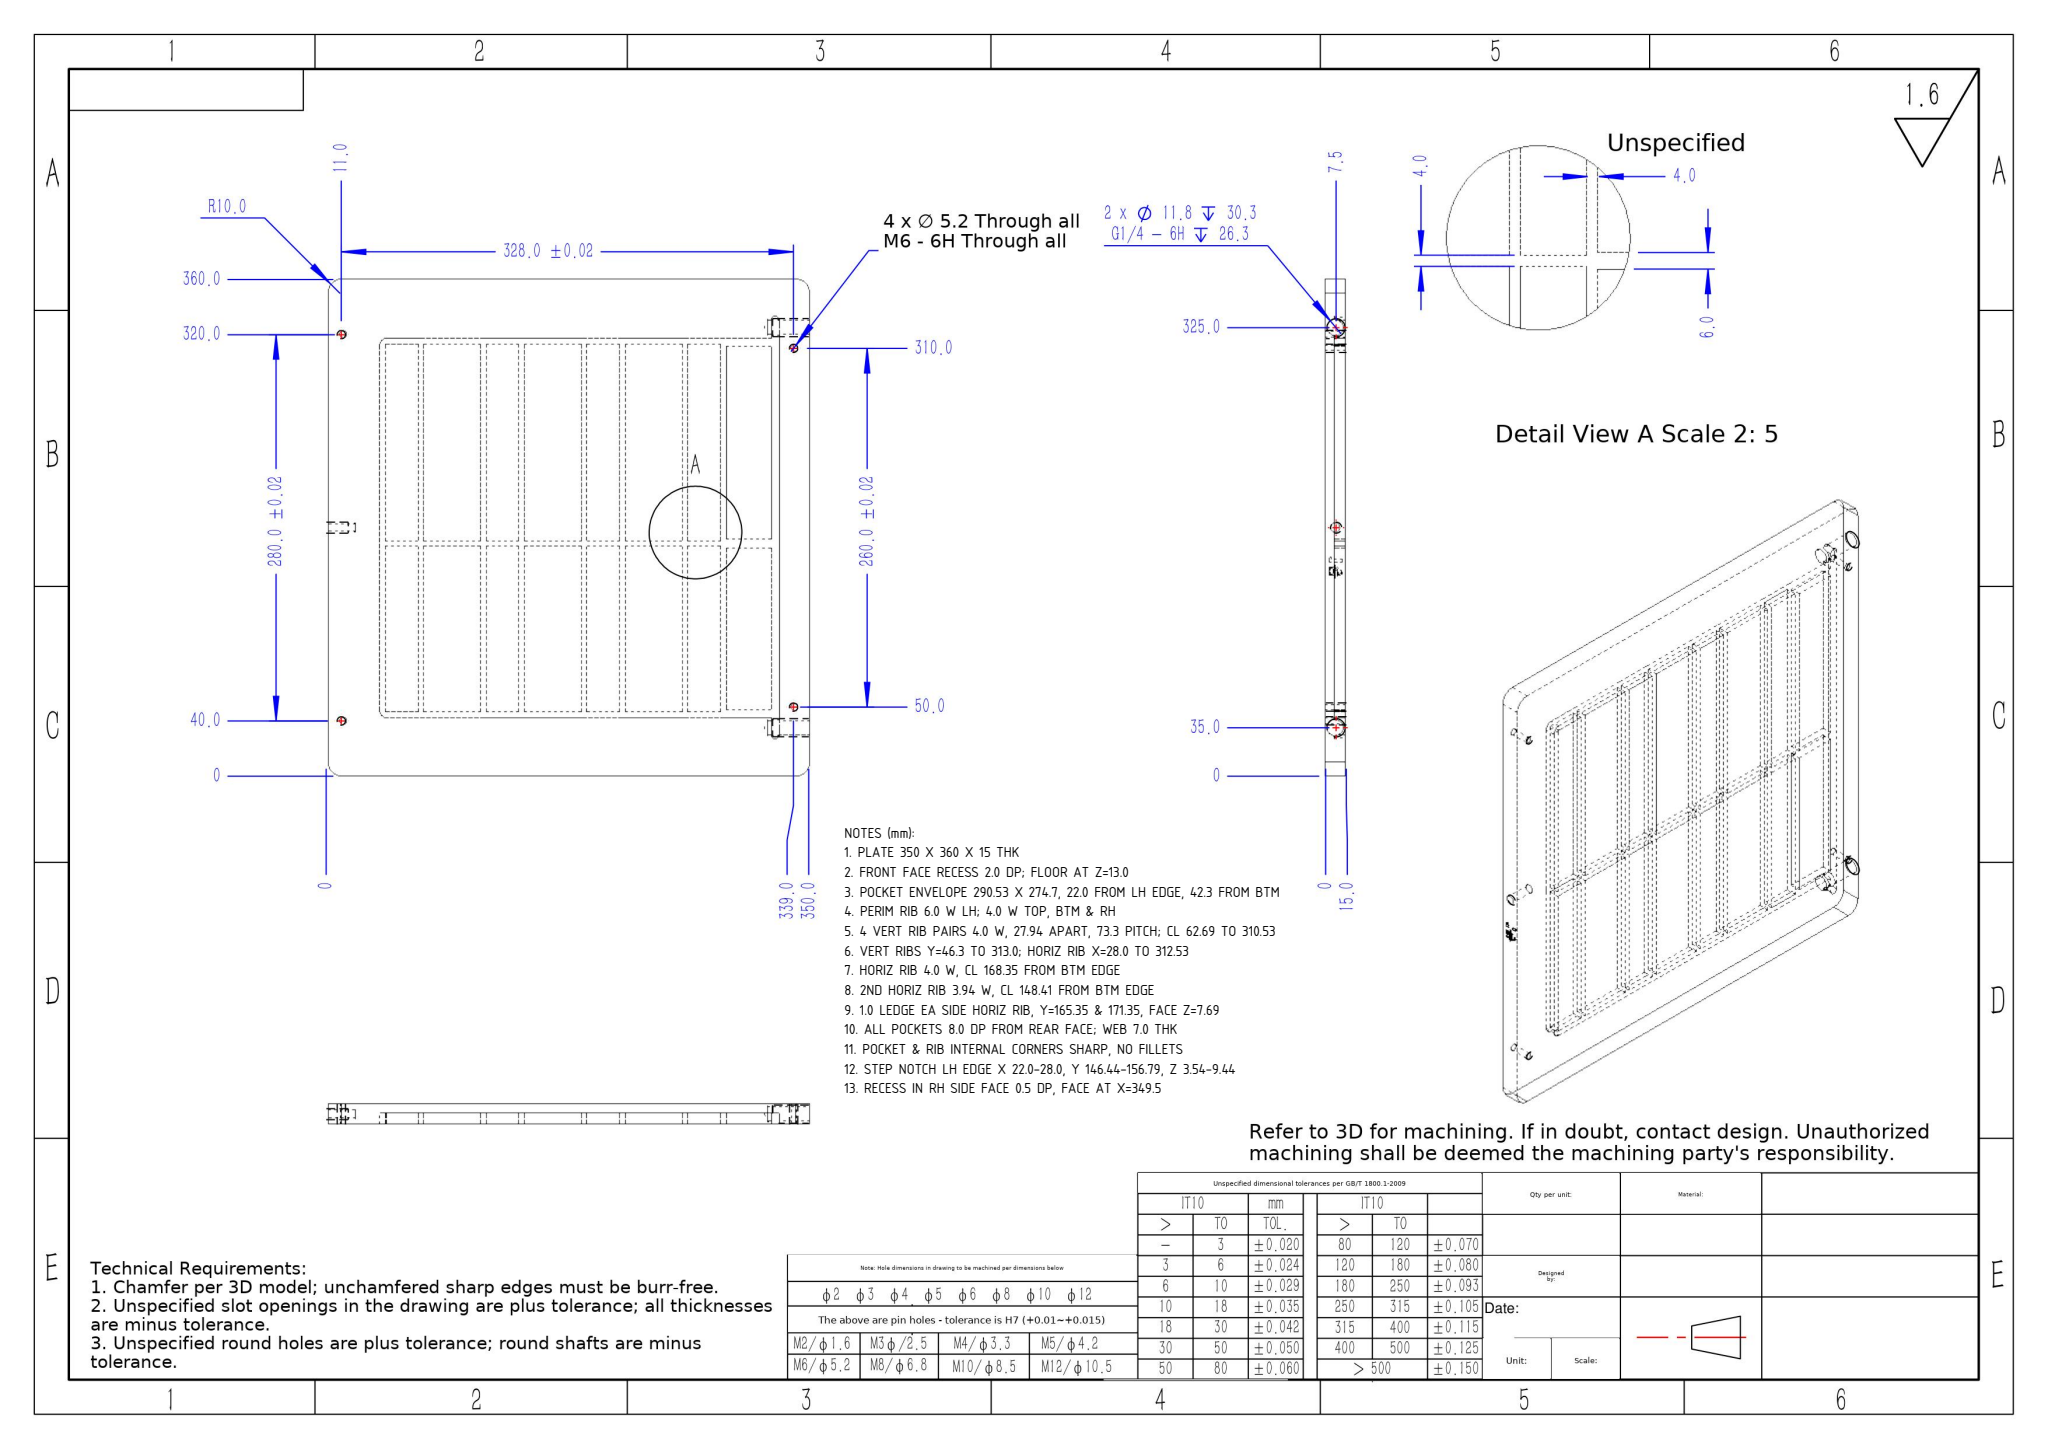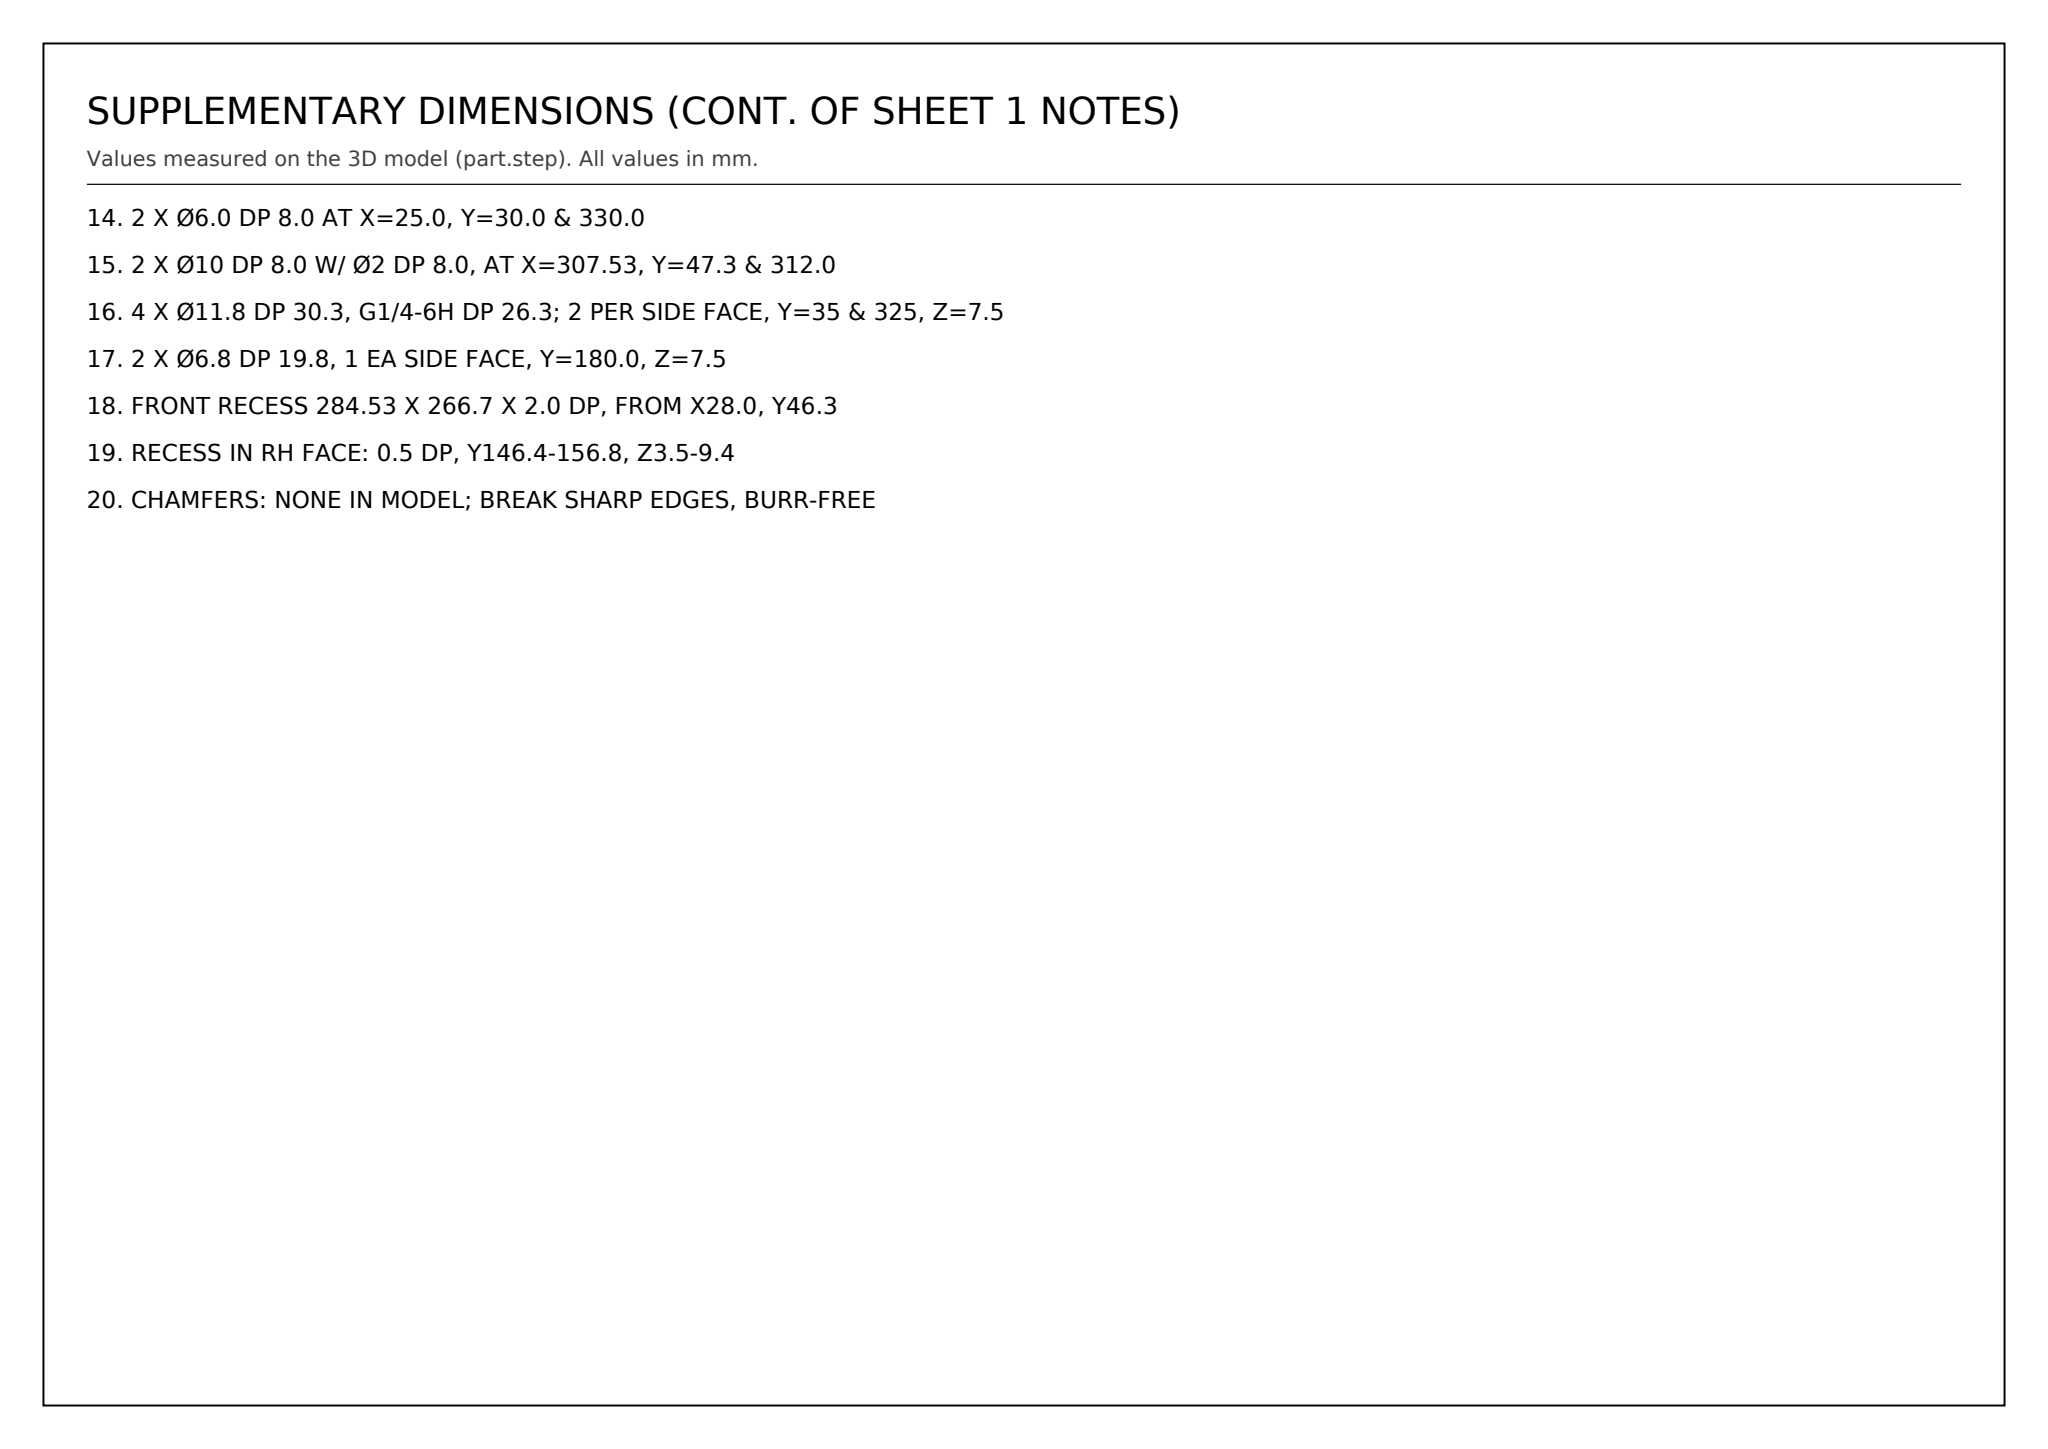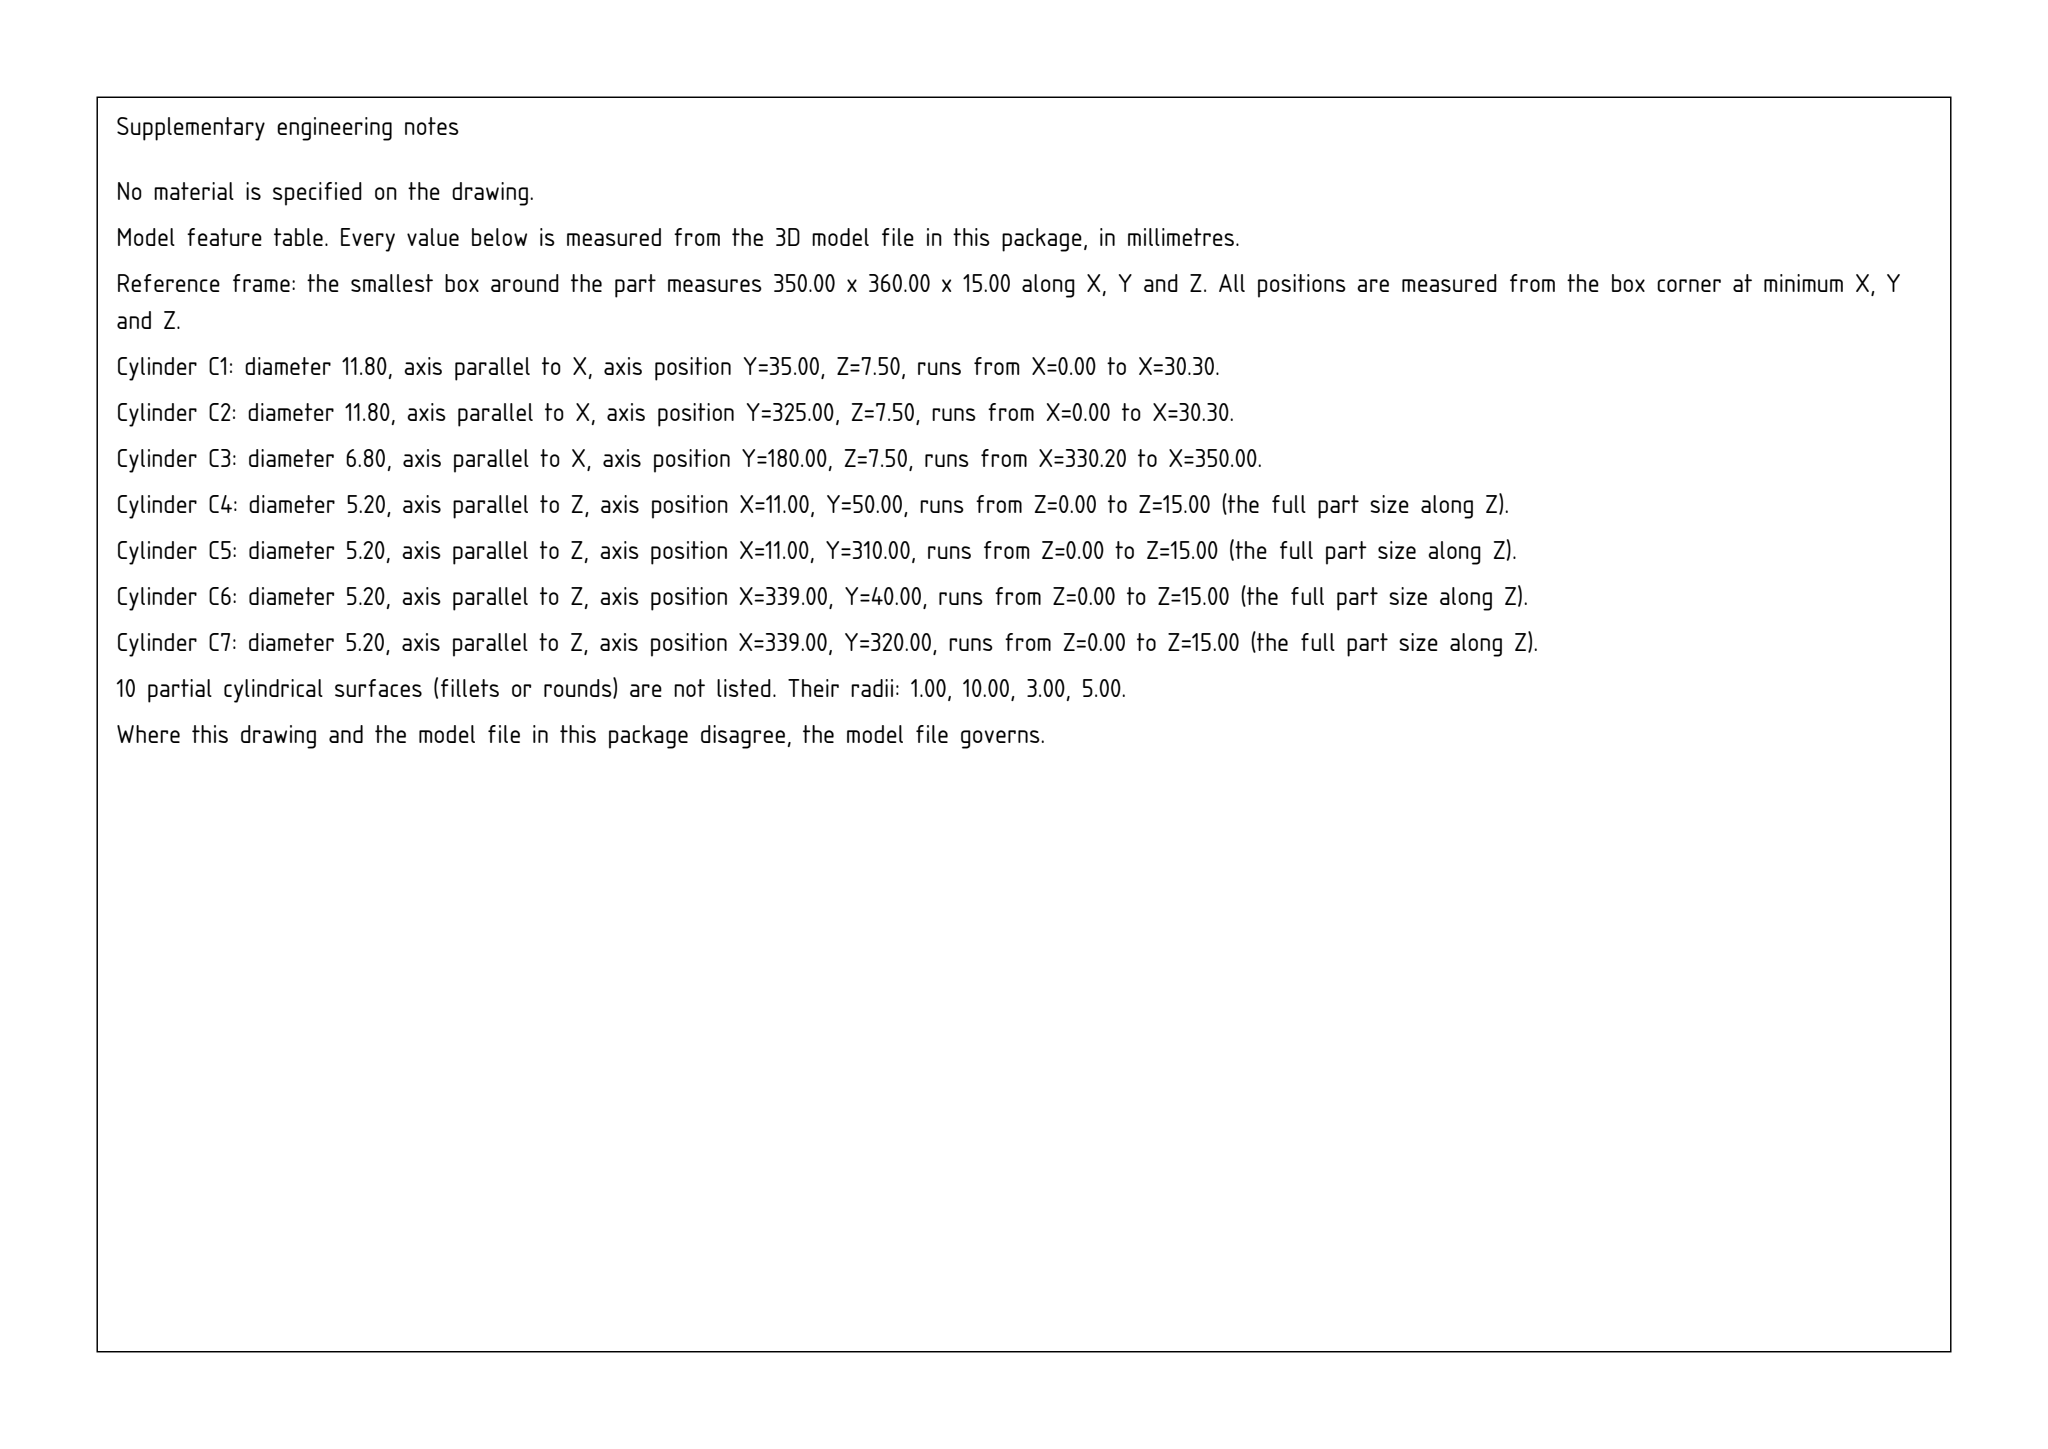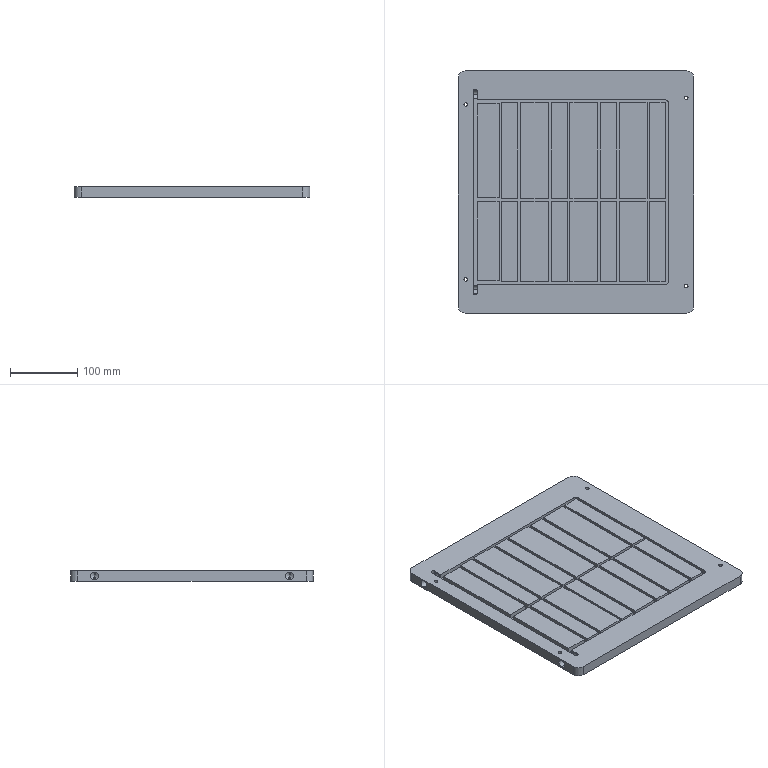Part | SolidWorks | mm | 1 solid | 172 faces | box 350 x 360 x 15 mm | volume 1769835 mm3 | plane 135 | cylinder 24 | spline 7 | cone 6 | commonest cylinder face diameters 5.2 x8 11.8 x4 20 x4 6.8 x2 10 x2 2 x2 6 x2
Drawing notes:
PLATE 350 X 360 X 15 THK | from the solid: bbox_xyz 350.0 x 360.0 x 15.0
FRONT FACE RECESS 2.0 DP; FLOOR AT Z=13.0 | from the solid: z plane 13.0 vs front face z 15.0
POCKET ENVELOPE 290.53 X 274.7, 22.0 FROM LH EDGE, 42.3 FROM BTM | from the solid: x 22.0 to 312.53 = 290.53; y 42.3 to 317.0 = 274.7
PERIM RIB 6.0 W LH; 4.0 W TOP, BTM & RH | from the solid: x 22.0-28.0 = 6.0; y 42.3-46.3 and 313.0-317.0 = 4.0; x 308.53-312.53 = 4.0
4 VERT RIB PAIRS 4.0 W, 27.94 APART, 73.3 PITCH; CL 62.69 TO 310.53 | from the solid: x faces 60.69/64.69, 88.63/92.63, 133.99/137.99, 161.93/165.93, 207.29/211.29, 235.23/239.23, 280.59/284.59, 308.53/312.53
VERT RIBS Y=46.3 TO 313.0; HORIZ RIB X=28.0 TO 312.53 | from the solid: y planes 46.3 & 313.0 (count 7 ea); x planes 28.0 & 312.53
HORIZ RIB 4.0 W, CL 168.35 FROM BTM EDGE | from the solid: y planes 166.35-170.35 = 4.0, CL 168.35
2ND HORIZ RIB 3.94 W, CL 148.41 FROM BTM EDGE | from the solid: y planes 146.44 & 150.38 (pair)
1.0 LEDGE EA SIDE HORIZ RIB, Y=165.35 & 171.35, FACE Z=7.69 | from the solid: y planes 165.35, 166.35, 170.35, 171.35; z faces 7.69 count 2 vs pocket floor 7.0
ALL POCKETS 8.0 DP FROM REAR FACE; WEB 7.0 THK | from the solid: z planes 7.0 (pocket floor) and 15.0 (face); plate thk 15.0
POCKET & RIB INTERNAL CORNERS SHARP, NO FILLETS | from the solid: fillet_radii: [] (no fillets in model)
STEP NOTCH LH EDGE X 22.0-28.0, Y 146.44-156.79, Z 3.54-9.44 | from the solid: x planes 22.0 & 28.0; y 146.44/150.38/155.0/156.79; z 3.54,4.67,5.9,6.36,7.23,7.69,8.98,9.44
RECESS IN RH SIDE FACE 0.5 DP, FACE AT X=349.5 | from the solid: axis_planes x 349.5 count 3 vs outer face x 350.0
2 X Ø6.0 DP 8.0 AT X=25.0, Y=30.0 & 330.0 | from the solid: cyl dia6.0 axis z, len 8.0 at (25,30) and (25,330)
2 X Ø10 DP 8.0 W/ Ø2 DP 8.0, AT X=307.53, Y=47.3 & 312.0 | from the solid: cyl dia10 z len8 and dia2 z len8 at (307.53,47.3) and (307.53,312.0)
4 X Ø11.8 DP 30.3, G1/4-6H DP 26.3; 2 PER SIDE FACE, Y=35 & 325, Z=7.5 | from the solid: cyl dia11.8 axis x at y=35 count 2 and y=325 count 2, z=7.5, L=30.3; cone 118 deg ref 11.8
2 X Ø6.8 DP 19.8, 1 EA SIDE FACE, Y=180.0, Z=7.5 | from the solid: cyl dia6.8 axis x, len 19.8, y=180.0 z=7.5, count 2, 118 deg point
FRONT RECESS 284.53 X 266.7 X 2.0 DP, FROM X28.0, Y46.3 | from the solid: z plane 13.0 (=15.0-2.0); pocket walls x=28.0 to 312.53, y=46.3 to 313.0
RECESS IN RH FACE: 0.5 DP, Y146.4-156.8, Z3.5-9.4 | from the solid: x plane 349.5 (0.5 below face x=350.0); y 146.44/156.79, z 3.54/9.44
CHAMFERS: NONE IN MODEL; BREAK SHARP EDGES, BURR-FREE | from the solid: no chamfer faces: fillet_radii empty; only 118 deg cones = drill points